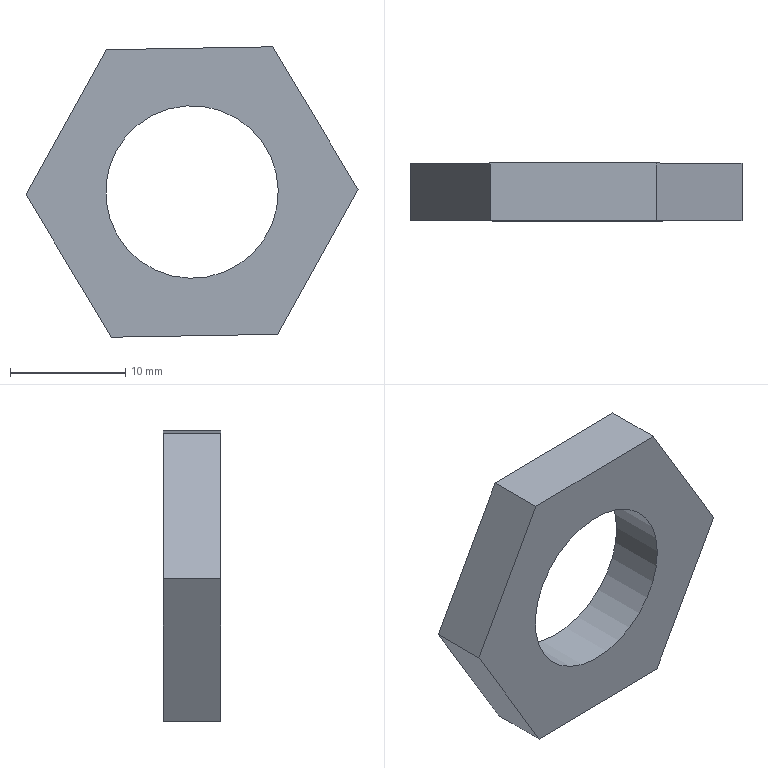Component | NX | NUT | 1 solid | 9 faces | box 28.86 x 5 x 25.25 mm | volume 1823 mm3 | plane 8 | cylinder 1 | commonest cylinder face diameters 15 x1
STEP:
#1=CARTESIAN_POINT('',(0.,0.,0.));
#2=DIRECTION('',(0.,0.,1.));
#3=DIRECTION('',(1.,0.,0.));
#4=AXIS2_PLACEMENT_3D('',#1,#2,#3);
#5=CARTESIAN_POINT('',(98.43,32.126,992.372));
#6=VERTEX_POINT('',#5);
#7=CARTESIAN_POINT('',(91.432,32.126,979.748));
#8=VERTEX_POINT('',#7);
#9=CARTESIAN_POINT('',(98.43,32.126,992.372));
#10=DIRECTION('',(-0.4848,0.,-0.8746));
#11=VECTOR('',#10,1.);
#12=LINE('',#9,#11);
#13=CARTESIAN_POINT('',(98.43,27.126,992.372));
#14=DIRECTION('',(0.8746,0.,-0.4848));
#15=DIRECTION('',(0.4848,0.,0.8746));
#16=AXIS2_PLACEMENT_3D('',#13,#14,#15);
#17=PLANE('',#16);
#18=CARTESIAN_POINT('',(0.,-5.));
#19=DIRECTION('',(-1.,0.));
#20=VECTOR('',#19,1.);
#21=LINE('',#18,#20);
#22=(GEOMETRIC_REPRESENTATION_CONTEXT(2)PARAMETRIC_REPRESENTATION_CONTEXT()REPRESENTATION_CONTEXT('',''));
#23=DEFINITIONAL_REPRESENTATION('',(#21),#22);
#24=PCURVE('',#17,#23);
#25=CARTESIAN_POINT('',(105.864,32.126,980.));
#26=DIRECTION('',(0.,-1.,0.));
#27=DIRECTION('',(1.,0.,0.));
#28=AXIS2_PLACEMENT_3D('',#25,#26,#27);
#29=PLANE('',#28);
#30=CARTESIAN_POINT('',(-7.434,12.372));
#31=DIRECTION('',(-0.4848,-0.8746));
#32=VECTOR('',#31,1.);
#33=LINE('',#30,#32);
#34=(GEOMETRIC_REPRESENTATION_CONTEXT(2)PARAMETRIC_REPRESENTATION_CONTEXT()REPRESENTATION_CONTEXT('',''));
#35=DEFINITIONAL_REPRESENTATION('',(#33),#34);
#36=PCURVE('',#29,#35);
#37=SURFACE_CURVE('',#12,(#24,#36),.PCURVE_S1.);
#38=EDGE_CURVE('',#6,#8,#37,.T.);
#39=ORIENTED_EDGE('',*,*,#38,.T.);
#40=CARTESIAN_POINT('',(91.432,27.126,979.748));
#41=VERTEX_POINT('',#40);
#42=CARTESIAN_POINT('',(91.432,27.126,979.748));
#43=DIRECTION('',(0.,1.,0.));
#44=VECTOR('',#43,1.);
#45=LINE('',#42,#44);
#46=CARTESIAN_POINT('',(-14.434,0.));
#47=DIRECTION('',(0.,-1.));
#48=VECTOR('',#47,1.);
#49=LINE('',#46,#48);
#50=(GEOMETRIC_REPRESENTATION_CONTEXT(2)PARAMETRIC_REPRESENTATION_CONTEXT()REPRESENTATION_CONTEXT('',''));
#51=DEFINITIONAL_REPRESENTATION('',(#49),#50);
#52=PCURVE('',#17,#51);
#53=CARTESIAN_POINT('',(91.432,27.126,979.748));
#54=DIRECTION('',(0.8572,0.,0.515));
#55=DIRECTION('',(-0.515,0.,0.8572));
#56=AXIS2_PLACEMENT_3D('',#53,#54,#55);
#57=PLANE('',#56);
#58=CARTESIAN_POINT('',(0.,0.));
#59=DIRECTION('',(0.,-1.));
#60=VECTOR('',#59,1.);
#61=LINE('',#58,#60);
#62=(GEOMETRIC_REPRESENTATION_CONTEXT(2)PARAMETRIC_REPRESENTATION_CONTEXT()REPRESENTATION_CONTEXT('',''));
#63=DEFINITIONAL_REPRESENTATION('',(#61),#62);
#64=PCURVE('',#57,#63);
#65=SURFACE_CURVE('',#45,(#52,#64),.PCURVE_S1.);
#66=EDGE_CURVE('',#41,#8,#65,.T.);
#67=ORIENTED_EDGE('',*,*,#66,.F.);
#68=CARTESIAN_POINT('',(98.43,27.126,992.372));
#69=VERTEX_POINT('',#68);
#70=CARTESIAN_POINT('',(98.43,27.126,992.372));
#71=DIRECTION('',(-0.4848,0.,-0.8746));
#72=VECTOR('',#71,1.);
#73=LINE('',#70,#72);
#74=CARTESIAN_POINT('',(0.,0.));
#75=DIRECTION('',(-1.,0.));
#76=VECTOR('',#75,1.);
#77=LINE('',#74,#76);
#78=(GEOMETRIC_REPRESENTATION_CONTEXT(2)PARAMETRIC_REPRESENTATION_CONTEXT()REPRESENTATION_CONTEXT('',''));
#79=DEFINITIONAL_REPRESENTATION('',(#77),#78);
#80=PCURVE('',#17,#79);
#81=CARTESIAN_POINT('',(105.864,27.126,980.));
#82=DIRECTION('',(0.,-1.,0.));
#83=DIRECTION('',(1.,0.,0.));
#84=AXIS2_PLACEMENT_3D('',#81,#82,#83);
#85=PLANE('',#84);
#86=CARTESIAN_POINT('',(-7.434,12.372));
#87=DIRECTION('',(-0.4848,-0.8746));
#88=VECTOR('',#87,1.);
#89=LINE('',#86,#88);
#90=(GEOMETRIC_REPRESENTATION_CONTEXT(2)PARAMETRIC_REPRESENTATION_CONTEXT()REPRESENTATION_CONTEXT('',''));
#91=DEFINITIONAL_REPRESENTATION('',(#89),#90);
#92=PCURVE('',#85,#91);
#93=SURFACE_CURVE('',#73,(#80,#92),.PCURVE_S1.);
#94=EDGE_CURVE('',#69,#41,#93,.T.);
#95=ORIENTED_EDGE('',*,*,#94,.F.);
#96=CARTESIAN_POINT('',(98.43,27.126,992.372));
#97=DIRECTION('',(0.,1.,0.));
#98=VECTOR('',#97,1.);
#99=LINE('',#96,#98);
#100=CARTESIAN_POINT('',(0.,0.));
#101=DIRECTION('',(0.,-1.));
#102=VECTOR('',#101,1.);
#103=LINE('',#100,#102);
#104=(GEOMETRIC_REPRESENTATION_CONTEXT(2)PARAMETRIC_REPRESENTATION_CONTEXT()REPRESENTATION_CONTEXT('',''));
#105=DEFINITIONAL_REPRESENTATION('',(#103),#104);
#106=PCURVE('',#17,#105);
#107=CARTESIAN_POINT('',(112.862,27.126,992.624));
#108=DIRECTION('',(0.01745,0.,-0.9998));
#109=DIRECTION('',(0.9998,0.,0.01745));
#110=AXIS2_PLACEMENT_3D('',#107,#108,#109);
#111=PLANE('',#110);
#112=CARTESIAN_POINT('',(-14.434,0.));
#113=DIRECTION('',(0.,-1.));
#114=VECTOR('',#113,1.);
#115=LINE('',#112,#114);
#116=(GEOMETRIC_REPRESENTATION_CONTEXT(2)PARAMETRIC_REPRESENTATION_CONTEXT()REPRESENTATION_CONTEXT('',''));
#117=DEFINITIONAL_REPRESENTATION('',(#115),#116);
#118=PCURVE('',#111,#117);
#119=SURFACE_CURVE('',#99,(#106,#118),.PCURVE_S1.);
#120=EDGE_CURVE('',#69,#6,#119,.T.);
#121=ORIENTED_EDGE('',*,*,#120,.T.);
#122=EDGE_LOOP('',(#39,#67,#95,#121));
#123=FACE_BOUND('',#122,.T.);
#124=ADVANCED_FACE('',(#123),#17,.F.);
#125=CARTESIAN_POINT('',(98.866,32.126,967.376));
#126=VERTEX_POINT('',#125);
#127=CARTESIAN_POINT('',(91.432,32.126,979.748));
#128=DIRECTION('',(0.515,0.,-0.8572));
#129=VECTOR('',#128,1.);
#130=LINE('',#127,#129);
#131=CARTESIAN_POINT('',(0.,-5.));
#132=DIRECTION('',(-1.,0.));
#133=VECTOR('',#132,1.);
#134=LINE('',#131,#133);
#135=(GEOMETRIC_REPRESENTATION_CONTEXT(2)PARAMETRIC_REPRESENTATION_CONTEXT()REPRESENTATION_CONTEXT('',''));
#136=DEFINITIONAL_REPRESENTATION('',(#134),#135);
#137=PCURVE('',#57,#136);
#138=CARTESIAN_POINT('',(-14.432,-0.2519));
#139=DIRECTION('',(0.515,-0.8572));
#140=VECTOR('',#139,1.);
#141=LINE('',#138,#140);
#142=(GEOMETRIC_REPRESENTATION_CONTEXT(2)PARAMETRIC_REPRESENTATION_CONTEXT()REPRESENTATION_CONTEXT('',''));
#143=DEFINITIONAL_REPRESENTATION('',(#141),#142);
#144=PCURVE('',#29,#143);
#145=SURFACE_CURVE('',#130,(#137,#144),.PCURVE_S1.);
#146=EDGE_CURVE('',#8,#126,#145,.T.);
#147=ORIENTED_EDGE('',*,*,#146,.T.);
#148=CARTESIAN_POINT('',(98.866,27.126,967.376));
#149=VERTEX_POINT('',#148);
#150=CARTESIAN_POINT('',(98.866,27.126,967.376));
#151=DIRECTION('',(0.,1.,0.));
#152=VECTOR('',#151,1.);
#153=LINE('',#150,#152);
#154=CARTESIAN_POINT('',(-14.434,0.));
#155=DIRECTION('',(0.,-1.));
#156=VECTOR('',#155,1.);
#157=LINE('',#154,#156);
#158=(GEOMETRIC_REPRESENTATION_CONTEXT(2)PARAMETRIC_REPRESENTATION_CONTEXT()REPRESENTATION_CONTEXT('',''));
#159=DEFINITIONAL_REPRESENTATION('',(#157),#158);
#160=PCURVE('',#57,#159);
#161=CARTESIAN_POINT('',(98.866,27.126,967.376));
#162=DIRECTION('',(-0.01745,0.,0.9998));
#163=DIRECTION('',(-0.9998,0.,-0.01745));
#164=AXIS2_PLACEMENT_3D('',#161,#162,#163);
#165=PLANE('',#164);
#166=CARTESIAN_POINT('',(0.,0.));
#167=DIRECTION('',(0.,-1.));
#168=VECTOR('',#167,1.);
#169=LINE('',#166,#168);
#170=(GEOMETRIC_REPRESENTATION_CONTEXT(2)PARAMETRIC_REPRESENTATION_CONTEXT()REPRESENTATION_CONTEXT('',''));
#171=DEFINITIONAL_REPRESENTATION('',(#169),#170);
#172=PCURVE('',#165,#171);
#173=SURFACE_CURVE('',#153,(#160,#172),.PCURVE_S1.);
#174=EDGE_CURVE('',#149,#126,#173,.T.);
#175=ORIENTED_EDGE('',*,*,#174,.F.);
#176=CARTESIAN_POINT('',(91.432,27.126,979.748));
#177=DIRECTION('',(0.515,0.,-0.8572));
#178=VECTOR('',#177,1.);
#179=LINE('',#176,#178);
#180=CARTESIAN_POINT('',(0.,0.));
#181=DIRECTION('',(-1.,0.));
#182=VECTOR('',#181,1.);
#183=LINE('',#180,#182);
#184=(GEOMETRIC_REPRESENTATION_CONTEXT(2)PARAMETRIC_REPRESENTATION_CONTEXT()REPRESENTATION_CONTEXT('',''));
#185=DEFINITIONAL_REPRESENTATION('',(#183),#184);
#186=PCURVE('',#57,#185);
#187=CARTESIAN_POINT('',(-14.432,-0.2519));
#188=DIRECTION('',(0.515,-0.8572));
#189=VECTOR('',#188,1.);
#190=LINE('',#187,#189);
#191=(GEOMETRIC_REPRESENTATION_CONTEXT(2)PARAMETRIC_REPRESENTATION_CONTEXT()REPRESENTATION_CONTEXT('',''));
#192=DEFINITIONAL_REPRESENTATION('',(#190),#191);
#193=PCURVE('',#85,#192);
#194=SURFACE_CURVE('',#179,(#186,#193),.PCURVE_S1.);
#195=EDGE_CURVE('',#41,#149,#194,.T.);
#196=ORIENTED_EDGE('',*,*,#195,.F.);
#197=ORIENTED_EDGE('',*,*,#66,.T.);
#198=EDGE_LOOP('',(#147,#175,#196,#197));
#199=FACE_BOUND('',#198,.T.);
#200=ADVANCED_FACE('',(#199),#57,.F.);
#201=CARTESIAN_POINT('',(113.298,32.126,967.628));
#202=VERTEX_POINT('',#201);
#203=CARTESIAN_POINT('',(98.866,32.126,967.376));
#204=DIRECTION('',(0.9998,0.,0.01745));
#205=VECTOR('',#204,1.);
#206=LINE('',#203,#205);
#207=CARTESIAN_POINT('',(0.,-5.));
#208=DIRECTION('',(-1.,0.));
#209=VECTOR('',#208,1.);
#210=LINE('',#207,#209);
#211=(GEOMETRIC_REPRESENTATION_CONTEXT(2)PARAMETRIC_REPRESENTATION_CONTEXT()REPRESENTATION_CONTEXT('',''));
#212=DEFINITIONAL_REPRESENTATION('',(#210),#211);
#213=PCURVE('',#165,#212);
#214=CARTESIAN_POINT('',(-6.998,-12.624));
#215=DIRECTION('',(0.9998,0.01745));
#216=VECTOR('',#215,1.);
#217=LINE('',#214,#216);
#218=(GEOMETRIC_REPRESENTATION_CONTEXT(2)PARAMETRIC_REPRESENTATION_CONTEXT()REPRESENTATION_CONTEXT('',''));
#219=DEFINITIONAL_REPRESENTATION('',(#217),#218);
#220=PCURVE('',#29,#219);
#221=SURFACE_CURVE('',#206,(#213,#220),.PCURVE_S1.);
#222=EDGE_CURVE('',#126,#202,#221,.T.);
#223=ORIENTED_EDGE('',*,*,#222,.T.);
#224=CARTESIAN_POINT('',(113.298,27.126,967.628));
#225=VERTEX_POINT('',#224);
#226=CARTESIAN_POINT('',(113.298,27.126,967.628));
#227=DIRECTION('',(0.,1.,0.));
#228=VECTOR('',#227,1.);
#229=LINE('',#226,#228);
#230=CARTESIAN_POINT('',(-14.434,0.));
#231=DIRECTION('',(0.,-1.));
#232=VECTOR('',#231,1.);
#233=LINE('',#230,#232);
#234=(GEOMETRIC_REPRESENTATION_CONTEXT(2)PARAMETRIC_REPRESENTATION_CONTEXT()REPRESENTATION_CONTEXT('',''));
#235=DEFINITIONAL_REPRESENTATION('',(#233),#234);
#236=PCURVE('',#165,#235);
#237=CARTESIAN_POINT('',(113.298,27.126,967.628));
#238=DIRECTION('',(-0.8746,0.,0.4848));
#239=DIRECTION('',(-0.4848,0.,-0.8746));
#240=AXIS2_PLACEMENT_3D('',#237,#238,#239);
#241=PLANE('',#240);
#242=CARTESIAN_POINT('',(0.,0.));
#243=DIRECTION('',(0.,-1.));
#244=VECTOR('',#243,1.);
#245=LINE('',#242,#244);
#246=(GEOMETRIC_REPRESENTATION_CONTEXT(2)PARAMETRIC_REPRESENTATION_CONTEXT()REPRESENTATION_CONTEXT('',''));
#247=DEFINITIONAL_REPRESENTATION('',(#245),#246);
#248=PCURVE('',#241,#247);
#249=SURFACE_CURVE('',#229,(#236,#248),.PCURVE_S1.);
#250=EDGE_CURVE('',#225,#202,#249,.T.);
#251=ORIENTED_EDGE('',*,*,#250,.F.);
#252=CARTESIAN_POINT('',(98.866,27.126,967.376));
#253=DIRECTION('',(0.9998,0.,0.01745));
#254=VECTOR('',#253,1.);
#255=LINE('',#252,#254);
#256=CARTESIAN_POINT('',(0.,0.));
#257=DIRECTION('',(-1.,0.));
#258=VECTOR('',#257,1.);
#259=LINE('',#256,#258);
#260=(GEOMETRIC_REPRESENTATION_CONTEXT(2)PARAMETRIC_REPRESENTATION_CONTEXT()REPRESENTATION_CONTEXT('',''));
#261=DEFINITIONAL_REPRESENTATION('',(#259),#260);
#262=PCURVE('',#165,#261);
#263=CARTESIAN_POINT('',(-6.998,-12.624));
#264=DIRECTION('',(0.9998,0.01745));
#265=VECTOR('',#264,1.);
#266=LINE('',#263,#265);
#267=(GEOMETRIC_REPRESENTATION_CONTEXT(2)PARAMETRIC_REPRESENTATION_CONTEXT()REPRESENTATION_CONTEXT('',''));
#268=DEFINITIONAL_REPRESENTATION('',(#266),#267);
#269=PCURVE('',#85,#268);
#270=SURFACE_CURVE('',#255,(#262,#269),.PCURVE_S1.);
#271=EDGE_CURVE('',#149,#225,#270,.T.);
#272=ORIENTED_EDGE('',*,*,#271,.F.);
#273=ORIENTED_EDGE('',*,*,#174,.T.);
#274=EDGE_LOOP('',(#223,#251,#272,#273));
#275=FACE_BOUND('',#274,.T.);
#276=ADVANCED_FACE('',(#275),#165,.F.);
#277=CARTESIAN_POINT('',(120.296,32.126,980.252));
#278=VERTEX_POINT('',#277);
#279=CARTESIAN_POINT('',(113.298,32.126,967.628));
#280=DIRECTION('',(0.4848,0.,0.8746));
#281=VECTOR('',#280,1.);
#282=LINE('',#279,#281);
#283=CARTESIAN_POINT('',(0.,-5.));
#284=DIRECTION('',(-1.,0.));
#285=VECTOR('',#284,1.);
#286=LINE('',#283,#285);
#287=(GEOMETRIC_REPRESENTATION_CONTEXT(2)PARAMETRIC_REPRESENTATION_CONTEXT()REPRESENTATION_CONTEXT('',''));
#288=DEFINITIONAL_REPRESENTATION('',(#286),#287);
#289=PCURVE('',#241,#288);
#290=CARTESIAN_POINT('',(7.434,-12.372));
#291=DIRECTION('',(0.4848,0.8746));
#292=VECTOR('',#291,1.);
#293=LINE('',#290,#292);
#294=(GEOMETRIC_REPRESENTATION_CONTEXT(2)PARAMETRIC_REPRESENTATION_CONTEXT()REPRESENTATION_CONTEXT('',''));
#295=DEFINITIONAL_REPRESENTATION('',(#293),#294);
#296=PCURVE('',#29,#295);
#297=SURFACE_CURVE('',#282,(#289,#296),.PCURVE_S1.);
#298=EDGE_CURVE('',#202,#278,#297,.T.);
#299=ORIENTED_EDGE('',*,*,#298,.T.);
#300=CARTESIAN_POINT('',(120.296,27.126,980.252));
#301=VERTEX_POINT('',#300);
#302=CARTESIAN_POINT('',(120.296,27.126,980.252));
#303=DIRECTION('',(0.,1.,0.));
#304=VECTOR('',#303,1.);
#305=LINE('',#302,#304);
#306=CARTESIAN_POINT('',(-14.434,0.));
#307=DIRECTION('',(0.,-1.));
#308=VECTOR('',#307,1.);
#309=LINE('',#306,#308);
#310=(GEOMETRIC_REPRESENTATION_CONTEXT(2)PARAMETRIC_REPRESENTATION_CONTEXT()REPRESENTATION_CONTEXT('',''));
#311=DEFINITIONAL_REPRESENTATION('',(#309),#310);
#312=PCURVE('',#241,#311);
#313=CARTESIAN_POINT('',(120.296,27.126,980.252));
#314=DIRECTION('',(-0.8572,0.,-0.515));
#315=DIRECTION('',(0.515,0.,-0.8572));
#316=AXIS2_PLACEMENT_3D('',#313,#314,#315);
#317=PLANE('',#316);
#318=CARTESIAN_POINT('',(0.,0.));
#319=DIRECTION('',(0.,-1.));
#320=VECTOR('',#319,1.);
#321=LINE('',#318,#320);
#322=(GEOMETRIC_REPRESENTATION_CONTEXT(2)PARAMETRIC_REPRESENTATION_CONTEXT()REPRESENTATION_CONTEXT('',''));
#323=DEFINITIONAL_REPRESENTATION('',(#321),#322);
#324=PCURVE('',#317,#323);
#325=SURFACE_CURVE('',#305,(#312,#324),.PCURVE_S1.);
#326=EDGE_CURVE('',#301,#278,#325,.T.);
#327=ORIENTED_EDGE('',*,*,#326,.F.);
#328=CARTESIAN_POINT('',(113.298,27.126,967.628));
#329=DIRECTION('',(0.4848,0.,0.8746));
#330=VECTOR('',#329,1.);
#331=LINE('',#328,#330);
#332=CARTESIAN_POINT('',(0.,0.));
#333=DIRECTION('',(-1.,0.));
#334=VECTOR('',#333,1.);
#335=LINE('',#332,#334);
#336=(GEOMETRIC_REPRESENTATION_CONTEXT(2)PARAMETRIC_REPRESENTATION_CONTEXT()REPRESENTATION_CONTEXT('',''));
#337=DEFINITIONAL_REPRESENTATION('',(#335),#336);
#338=PCURVE('',#241,#337);
#339=CARTESIAN_POINT('',(7.434,-12.372));
#340=DIRECTION('',(0.4848,0.8746));
#341=VECTOR('',#340,1.);
#342=LINE('',#339,#341);
#343=(GEOMETRIC_REPRESENTATION_CONTEXT(2)PARAMETRIC_REPRESENTATION_CONTEXT()REPRESENTATION_CONTEXT('',''));
#344=DEFINITIONAL_REPRESENTATION('',(#342),#343);
#345=PCURVE('',#85,#344);
#346=SURFACE_CURVE('',#331,(#338,#345),.PCURVE_S1.);
#347=EDGE_CURVE('',#225,#301,#346,.T.);
#348=ORIENTED_EDGE('',*,*,#347,.F.);
#349=ORIENTED_EDGE('',*,*,#250,.T.);
#350=EDGE_LOOP('',(#299,#327,#348,#349));
#351=FACE_BOUND('',#350,.T.);
#352=ADVANCED_FACE('',(#351),#241,.F.);
#353=CARTESIAN_POINT('',(112.862,32.126,992.624));
#354=VERTEX_POINT('',#353);
#355=CARTESIAN_POINT('',(120.296,32.126,980.252));
#356=DIRECTION('',(-0.515,0.,0.8572));
#357=VECTOR('',#356,1.);
#358=LINE('',#355,#357);
#359=CARTESIAN_POINT('',(0.,-5.));
#360=DIRECTION('',(-1.,0.));
#361=VECTOR('',#360,1.);
#362=LINE('',#359,#361);
#363=(GEOMETRIC_REPRESENTATION_CONTEXT(2)PARAMETRIC_REPRESENTATION_CONTEXT()REPRESENTATION_CONTEXT('',''));
#364=DEFINITIONAL_REPRESENTATION('',(#362),#363);
#365=PCURVE('',#317,#364);
#366=CARTESIAN_POINT('',(14.432,0.2519));
#367=DIRECTION('',(-0.515,0.8572));
#368=VECTOR('',#367,1.);
#369=LINE('',#366,#368);
#370=(GEOMETRIC_REPRESENTATION_CONTEXT(2)PARAMETRIC_REPRESENTATION_CONTEXT()REPRESENTATION_CONTEXT('',''));
#371=DEFINITIONAL_REPRESENTATION('',(#369),#370);
#372=PCURVE('',#29,#371);
#373=SURFACE_CURVE('',#358,(#365,#372),.PCURVE_S1.);
#374=EDGE_CURVE('',#278,#354,#373,.T.);
#375=ORIENTED_EDGE('',*,*,#374,.T.);
#376=CARTESIAN_POINT('',(112.862,27.126,992.624));
#377=VERTEX_POINT('',#376);
#378=CARTESIAN_POINT('',(112.862,27.126,992.624));
#379=DIRECTION('',(0.,1.,0.));
#380=VECTOR('',#379,1.);
#381=LINE('',#378,#380);
#382=CARTESIAN_POINT('',(-14.434,0.));
#383=DIRECTION('',(0.,-1.));
#384=VECTOR('',#383,1.);
#385=LINE('',#382,#384);
#386=(GEOMETRIC_REPRESENTATION_CONTEXT(2)PARAMETRIC_REPRESENTATION_CONTEXT()REPRESENTATION_CONTEXT('',''));
#387=DEFINITIONAL_REPRESENTATION('',(#385),#386);
#388=PCURVE('',#317,#387);
#389=CARTESIAN_POINT('',(0.,0.));
#390=DIRECTION('',(0.,-1.));
#391=VECTOR('',#390,1.);
#392=LINE('',#389,#391);
#393=(GEOMETRIC_REPRESENTATION_CONTEXT(2)PARAMETRIC_REPRESENTATION_CONTEXT()REPRESENTATION_CONTEXT('',''));
#394=DEFINITIONAL_REPRESENTATION('',(#392),#393);
#395=PCURVE('',#111,#394);
#396=SURFACE_CURVE('',#381,(#388,#395),.PCURVE_S1.);
#397=EDGE_CURVE('',#377,#354,#396,.T.);
#398=ORIENTED_EDGE('',*,*,#397,.F.);
#399=CARTESIAN_POINT('',(120.296,27.126,980.252));
#400=DIRECTION('',(-0.515,0.,0.8572));
#401=VECTOR('',#400,1.);
#402=LINE('',#399,#401);
#403=CARTESIAN_POINT('',(0.,0.));
#404=DIRECTION('',(-1.,0.));
#405=VECTOR('',#404,1.);
#406=LINE('',#403,#405);
#407=(GEOMETRIC_REPRESENTATION_CONTEXT(2)PARAMETRIC_REPRESENTATION_CONTEXT()REPRESENTATION_CONTEXT('',''));
#408=DEFINITIONAL_REPRESENTATION('',(#406),#407);
#409=PCURVE('',#317,#408);
#410=CARTESIAN_POINT('',(14.432,0.2519));
#411=DIRECTION('',(-0.515,0.8572));
#412=VECTOR('',#411,1.);
#413=LINE('',#410,#412);
#414=(GEOMETRIC_REPRESENTATION_CONTEXT(2)PARAMETRIC_REPRESENTATION_CONTEXT()REPRESENTATION_CONTEXT('',''));
#415=DEFINITIONAL_REPRESENTATION('',(#413),#414);
#416=PCURVE('',#85,#415);
#417=SURFACE_CURVE('',#402,(#409,#416),.PCURVE_S1.);
#418=EDGE_CURVE('',#301,#377,#417,.T.);
#419=ORIENTED_EDGE('',*,*,#418,.F.);
#420=ORIENTED_EDGE('',*,*,#326,.T.);
#421=EDGE_LOOP('',(#375,#398,#419,#420));
#422=FACE_BOUND('',#421,.T.);
#423=ADVANCED_FACE('',(#422),#317,.F.);
#424=CARTESIAN_POINT('',(112.862,32.126,992.624));
#425=DIRECTION('',(-0.9998,0.,-0.01745));
#426=VECTOR('',#425,1.);
#427=LINE('',#424,#426);
#428=CARTESIAN_POINT('',(0.,-5.));
#429=DIRECTION('',(-1.,0.));
#430=VECTOR('',#429,1.);
#431=LINE('',#428,#430);
#432=(GEOMETRIC_REPRESENTATION_CONTEXT(2)PARAMETRIC_REPRESENTATION_CONTEXT()REPRESENTATION_CONTEXT('',''));
#433=DEFINITIONAL_REPRESENTATION('',(#431),#432);
#434=PCURVE('',#111,#433);
#435=CARTESIAN_POINT('',(6.998,12.624));
#436=DIRECTION('',(-0.9998,-0.01745));
#437=VECTOR('',#436,1.);
#438=LINE('',#435,#437);
#439=(GEOMETRIC_REPRESENTATION_CONTEXT(2)PARAMETRIC_REPRESENTATION_CONTEXT()REPRESENTATION_CONTEXT('',''));
#440=DEFINITIONAL_REPRESENTATION('',(#438),#439);
#441=PCURVE('',#29,#440);
#442=SURFACE_CURVE('',#427,(#434,#441),.PCURVE_S1.);
#443=EDGE_CURVE('',#354,#6,#442,.T.);
#444=ORIENTED_EDGE('',*,*,#443,.T.);
#445=ORIENTED_EDGE('',*,*,#120,.F.);
#446=CARTESIAN_POINT('',(112.862,27.126,992.624));
#447=DIRECTION('',(-0.9998,0.,-0.01745));
#448=VECTOR('',#447,1.);
#449=LINE('',#446,#448);
#450=CARTESIAN_POINT('',(0.,0.));
#451=DIRECTION('',(-1.,0.));
#452=VECTOR('',#451,1.);
#453=LINE('',#450,#452);
#454=(GEOMETRIC_REPRESENTATION_CONTEXT(2)PARAMETRIC_REPRESENTATION_CONTEXT()REPRESENTATION_CONTEXT('',''));
#455=DEFINITIONAL_REPRESENTATION('',(#453),#454);
#456=PCURVE('',#111,#455);
#457=CARTESIAN_POINT('',(6.998,12.624));
#458=DIRECTION('',(-0.9998,-0.01745));
#459=VECTOR('',#458,1.);
#460=LINE('',#457,#459);
#461=(GEOMETRIC_REPRESENTATION_CONTEXT(2)PARAMETRIC_REPRESENTATION_CONTEXT()REPRESENTATION_CONTEXT('',''));
#462=DEFINITIONAL_REPRESENTATION('',(#460),#461);
#463=PCURVE('',#85,#462);
#464=SURFACE_CURVE('',#449,(#456,#463),.PCURVE_S1.);
#465=EDGE_CURVE('',#377,#69,#464,.T.);
#466=ORIENTED_EDGE('',*,*,#465,.F.);
#467=ORIENTED_EDGE('',*,*,#397,.T.);
#468=EDGE_LOOP('',(#444,#445,#466,#467));
#469=FACE_BOUND('',#468,.T.);
#470=ADVANCED_FACE('',(#469),#111,.F.);
#471=CARTESIAN_POINT('',(113.363,27.126,980.131));
#472=VERTEX_POINT('',#471);
#473=CARTESIAN_POINT('',(105.864,27.126,980.));
#474=DIRECTION('',(0.,-1.,0.));
#475=DIRECTION('',(0.9998,0.,0.01745));
#476=AXIS2_PLACEMENT_3D('',#473,#474,#475);
#477=CIRCLE('',#476,7.5);
#478=CARTESIAN_POINT('',(0.,0.));
#479=DIRECTION('',(0.9998,0.01745));
#480=AXIS2_PLACEMENT_2D('',#478,#479);
#481=CIRCLE('',#480,7.5);
#482=(GEOMETRIC_REPRESENTATION_CONTEXT(2)PARAMETRIC_REPRESENTATION_CONTEXT()REPRESENTATION_CONTEXT('',''));
#483=DEFINITIONAL_REPRESENTATION('',(#481),#482);
#484=PCURVE('',#85,#483);
#485=CARTESIAN_POINT('',(105.864,32.126,980.));
#486=DIRECTION('',(0.,-1.,0.));
#487=DIRECTION('',(1.,0.,0.));
#488=AXIS2_PLACEMENT_3D('',#485,#486,#487);
#489=CYLINDRICAL_SURFACE('',#488,7.5);
#490=CARTESIAN_POINT('',(0.01745,5.));
#491=DIRECTION('',(1.,0.));
#492=VECTOR('',#491,1.);
#493=LINE('',#490,#492);
#494=(GEOMETRIC_REPRESENTATION_CONTEXT(2)PARAMETRIC_REPRESENTATION_CONTEXT()REPRESENTATION_CONTEXT('',''));
#495=DEFINITIONAL_REPRESENTATION('',(#493),#494);
#496=PCURVE('',#489,#495);
#497=SURFACE_CURVE('',#477,(#484,#496),.PCURVE_S1.);
#498=EDGE_CURVE('',#472,#472,#497,.T.);
#499=ORIENTED_EDGE('',*,*,#498,.F.);
#500=EDGE_LOOP('',(#499));
#501=FACE_BOUND('',#500,.T.);
#502=ORIENTED_EDGE('',*,*,#94,.T.);
#503=ORIENTED_EDGE('',*,*,#195,.T.);
#504=ORIENTED_EDGE('',*,*,#271,.T.);
#505=ORIENTED_EDGE('',*,*,#347,.T.);
#506=ORIENTED_EDGE('',*,*,#418,.T.);
#507=ORIENTED_EDGE('',*,*,#465,.T.);
#508=EDGE_LOOP('',(#502,#503,#504,#505,#506,#507));
#509=FACE_BOUND('',#508,.T.);
#510=ADVANCED_FACE('',(#501,#509),#85,.T.);
#511=CARTESIAN_POINT('',(113.363,32.126,980.131));
#512=VERTEX_POINT('',#511);
#513=CARTESIAN_POINT('',(105.864,32.126,980.));
#514=DIRECTION('',(0.,-1.,0.));
#515=DIRECTION('',(0.9998,0.,0.01745));
#516=AXIS2_PLACEMENT_3D('',#513,#514,#515);
#517=CIRCLE('',#516,7.5);
#518=CARTESIAN_POINT('',(0.,0.));
#519=DIRECTION('',(0.9998,0.01745));
#520=AXIS2_PLACEMENT_2D('',#518,#519);
#521=CIRCLE('',#520,7.5);
#522=(GEOMETRIC_REPRESENTATION_CONTEXT(2)PARAMETRIC_REPRESENTATION_CONTEXT()REPRESENTATION_CONTEXT('',''));
#523=DEFINITIONAL_REPRESENTATION('',(#521),#522);
#524=PCURVE('',#29,#523);
#525=CARTESIAN_POINT('',(0.01745,0.));
#526=DIRECTION('',(1.,0.));
#527=VECTOR('',#526,1.);
#528=LINE('',#525,#527);
#529=(GEOMETRIC_REPRESENTATION_CONTEXT(2)PARAMETRIC_REPRESENTATION_CONTEXT()REPRESENTATION_CONTEXT('',''));
#530=DEFINITIONAL_REPRESENTATION('',(#528),#529);
#531=PCURVE('',#489,#530);
#532=SURFACE_CURVE('',#517,(#524,#531),.PCURVE_S1.);
#533=EDGE_CURVE('',#512,#512,#532,.T.);
#534=ORIENTED_EDGE('',*,*,#533,.T.);
#535=EDGE_LOOP('',(#534));
#536=FACE_BOUND('',#535,.T.);
#537=ORIENTED_EDGE('',*,*,#38,.F.);
#538=ORIENTED_EDGE('',*,*,#443,.F.);
#539=ORIENTED_EDGE('',*,*,#374,.F.);
#540=ORIENTED_EDGE('',*,*,#298,.F.);
#541=ORIENTED_EDGE('',*,*,#222,.F.);
#542=ORIENTED_EDGE('',*,*,#146,.F.);
#543=EDGE_LOOP('',(#537,#538,#539,#540,#541,#542));
#544=FACE_BOUND('',#543,.T.);
#545=ADVANCED_FACE('',(#536,#544),#29,.F.);
#546=ORIENTED_EDGE('',*,*,#533,.T.);
#547=CARTESIAN_POINT('',(113.363,32.126,980.131));
#548=CARTESIAN_POINT('',(113.363,27.126,980.131));
#549=B_SPLINE_CURVE_WITH_KNOTS('',1,(#547,#548),.UNSPECIFIED.,.F.,.F.,(2,2),(0.,5.),.PIECEWISE_BEZIER_KNOTS.);
#550=CARTESIAN_POINT('',(6.301,0.));
#551=DIRECTION('',(0.,1.));
#552=VECTOR('',#551,1.);
#553=LINE('',#550,#552);
#554=(GEOMETRIC_REPRESENTATION_CONTEXT(2)PARAMETRIC_REPRESENTATION_CONTEXT()REPRESENTATION_CONTEXT('',''));
#555=DEFINITIONAL_REPRESENTATION('',(#553),#554);
#556=PCURVE('',#489,#555);
#557=CARTESIAN_POINT('',(0.01745,0.));
#558=DIRECTION('',(0.,1.));
#559=VECTOR('',#558,1.);
#560=LINE('',#557,#559);
#561=(GEOMETRIC_REPRESENTATION_CONTEXT(2)PARAMETRIC_REPRESENTATION_CONTEXT()REPRESENTATION_CONTEXT('',''));
#562=DEFINITIONAL_REPRESENTATION('',(#560),#561);
#563=PCURVE('',#489,#562);
#564=SEAM_CURVE('',#549,(#556,#563),.PCURVE_S1.);
#565=EDGE_CURVE('',#512,#472,#564,.T.);
#566=ORIENTED_EDGE('',*,*,#565,.T.);
#567=ORIENTED_EDGE('',*,*,#498,.F.);
#568=ORIENTED_EDGE('',*,*,#565,.F.);
#569=EDGE_LOOP('',(#546,#566,#567,#568));
#570=FACE_BOUND('',#569,.F.);
#571=ADVANCED_FACE('',(#570),#489,.F.);
#572=CLOSED_SHELL('',(#124,#200,#276,#352,#423,#470,#510,#545,#571));
#573=MANIFOLD_SOLID_BREP('',#572);
#574=(LENGTH_UNIT()NAMED_UNIT(*)SI_UNIT(.MILLI.,.METRE.));
#575=UNCERTAINTY_MEASURE_WITH_UNIT(LENGTH_MEASURE(0.000001),#574,'','');
#576=(NAMED_UNIT(*)PLANE_ANGLE_UNIT()SI_UNIT($,.RADIAN.));
#577=(NAMED_UNIT(*)SI_UNIT($,.STERADIAN.)SOLID_ANGLE_UNIT());
#578=(GEOMETRIC_REPRESENTATION_CONTEXT(3)GLOBAL_UNCERTAINTY_ASSIGNED_CONTEXT((#575))GLOBAL_UNIT_ASSIGNED_CONTEXT((#574,#576,#577))REPRESENTATION_CONTEXT('',''));
#579=ADVANCED_BREP_SHAPE_REPRESENTATION('',(#4,#573),#578);